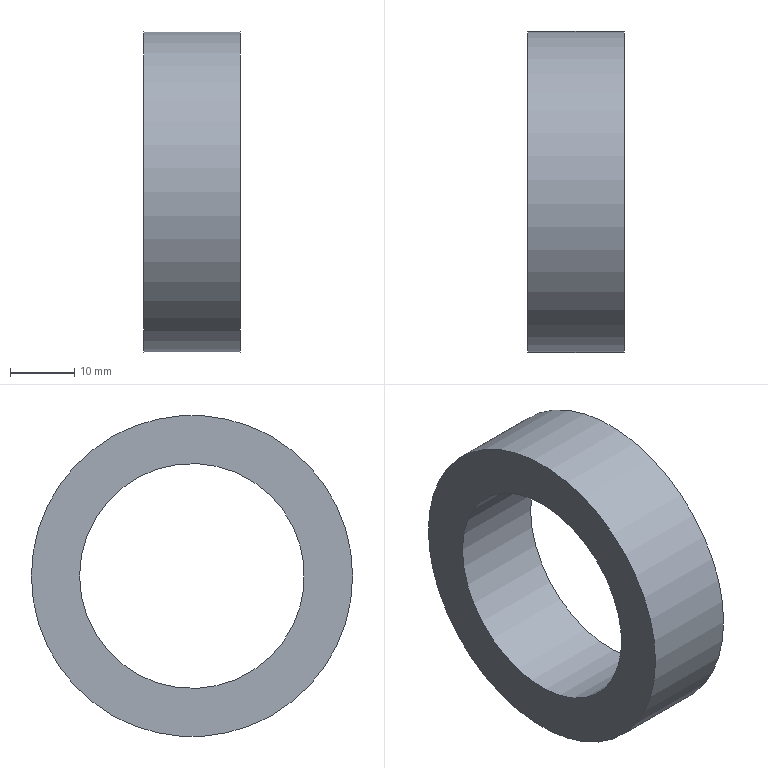Component | NX | CHENTAO | 1 solid | 4 faces | box 15 x 50 x 50 mm | volume 15021 mm3 | cylinder 2 | plane 2 | commonest cylinder face diameters 50 x1 35 x1
STEP:
#1=CARTESIAN_POINT('',(0.,0.,0.));
#2=DIRECTION('',(0.,0.,1.));
#3=DIRECTION('',(1.,0.,0.));
#4=AXIS2_PLACEMENT_3D('',#1,#2,#3);
#5=CARTESIAN_POINT('',(70.25,225.,-88.));
#6=VERTEX_POINT('',#5);
#7=CARTESIAN_POINT('',(70.25,200.,-88.));
#8=DIRECTION('',(1.,0.,0.));
#9=DIRECTION('',(0.,1.,0.));
#10=AXIS2_PLACEMENT_3D('',#7,#8,#9);
#11=CIRCLE('',#10,25.);
#12=CARTESIAN_POINT('',(70.25,200.,-88.));
#13=DIRECTION('',(-1.,0.,0.));
#14=DIRECTION('',(0.,0.,1.));
#15=AXIS2_PLACEMENT_3D('',#12,#13,#14);
#16=CYLINDRICAL_SURFACE('',#15,25.);
#17=CARTESIAN_POINT('',(7.854,0.));
#18=DIRECTION('',(-1.,0.));
#19=VECTOR('',#18,1.);
#20=LINE('',#17,#19);
#21=(GEOMETRIC_REPRESENTATION_CONTEXT(2)PARAMETRIC_REPRESENTATION_CONTEXT()REPRESENTATION_CONTEXT('',''));
#22=DEFINITIONAL_REPRESENTATION('',(#20),#21);
#23=PCURVE('',#16,#22);
#24=CARTESIAN_POINT('',(70.25,200.,-88.));
#25=DIRECTION('',(1.,0.,0.));
#26=DIRECTION('',(0.,0.,-1.));
#27=AXIS2_PLACEMENT_3D('',#24,#25,#26);
#28=PLANE('',#27);
#29=CARTESIAN_POINT('',(0.,0.));
#30=DIRECTION('',(0.,1.));
#31=AXIS2_PLACEMENT_2D('',#29,#30);
#32=CIRCLE('',#31,25.);
#33=(GEOMETRIC_REPRESENTATION_CONTEXT(2)PARAMETRIC_REPRESENTATION_CONTEXT()REPRESENTATION_CONTEXT('',''));
#34=DEFINITIONAL_REPRESENTATION('',(#32),#33);
#35=PCURVE('',#28,#34);
#36=SURFACE_CURVE('',#11,(#23,#35),.PCURVE_S1.);
#37=EDGE_CURVE('',#6,#6,#36,.T.);
#38=ORIENTED_EDGE('',*,*,#37,.F.);
#39=CARTESIAN_POINT('',(55.25,225.,-88.));
#40=VERTEX_POINT('',#39);
#41=CARTESIAN_POINT('',(70.25,225.,-88.));
#42=CARTESIAN_POINT('',(55.25,225.,-88.));
#43=B_SPLINE_CURVE_WITH_KNOTS('',1,(#41,#42),.UNSPECIFIED.,.F.,.F.,(2,2),(0.,15.),.PIECEWISE_BEZIER_KNOTS.);
#44=CARTESIAN_POINT('',(7.854,0.));
#45=DIRECTION('',(0.,1.));
#46=VECTOR('',#45,1.);
#47=LINE('',#44,#46);
#48=(GEOMETRIC_REPRESENTATION_CONTEXT(2)PARAMETRIC_REPRESENTATION_CONTEXT()REPRESENTATION_CONTEXT('',''));
#49=DEFINITIONAL_REPRESENTATION('',(#47),#48);
#50=PCURVE('',#16,#49);
#51=CARTESIAN_POINT('',(1.571,0.));
#52=DIRECTION('',(0.,1.));
#53=VECTOR('',#52,1.);
#54=LINE('',#51,#53);
#55=(GEOMETRIC_REPRESENTATION_CONTEXT(2)PARAMETRIC_REPRESENTATION_CONTEXT()REPRESENTATION_CONTEXT('',''));
#56=DEFINITIONAL_REPRESENTATION('',(#54),#55);
#57=PCURVE('',#16,#56);
#58=SEAM_CURVE('',#43,(#50,#57),.PCURVE_S1.);
#59=EDGE_CURVE('',#6,#40,#58,.T.);
#60=ORIENTED_EDGE('',*,*,#59,.T.);
#61=CARTESIAN_POINT('',(55.25,200.,-88.));
#62=DIRECTION('',(1.,0.,0.));
#63=DIRECTION('',(0.,1.,0.));
#64=AXIS2_PLACEMENT_3D('',#61,#62,#63);
#65=CIRCLE('',#64,25.);
#66=CARTESIAN_POINT('',(7.854,15.));
#67=DIRECTION('',(-1.,0.));
#68=VECTOR('',#67,1.);
#69=LINE('',#66,#68);
#70=(GEOMETRIC_REPRESENTATION_CONTEXT(2)PARAMETRIC_REPRESENTATION_CONTEXT()REPRESENTATION_CONTEXT('',''));
#71=DEFINITIONAL_REPRESENTATION('',(#69),#70);
#72=PCURVE('',#16,#71);
#73=CARTESIAN_POINT('',(55.25,200.,-88.));
#74=DIRECTION('',(1.,0.,0.));
#75=DIRECTION('',(0.,0.,-1.));
#76=AXIS2_PLACEMENT_3D('',#73,#74,#75);
#77=PLANE('',#76);
#78=CARTESIAN_POINT('',(0.,0.));
#79=DIRECTION('',(0.,1.));
#80=AXIS2_PLACEMENT_2D('',#78,#79);
#81=CIRCLE('',#80,25.);
#82=(GEOMETRIC_REPRESENTATION_CONTEXT(2)PARAMETRIC_REPRESENTATION_CONTEXT()REPRESENTATION_CONTEXT('',''));
#83=DEFINITIONAL_REPRESENTATION('',(#81),#82);
#84=PCURVE('',#77,#83);
#85=SURFACE_CURVE('',#65,(#72,#84),.PCURVE_S1.);
#86=EDGE_CURVE('',#40,#40,#85,.T.);
#87=ORIENTED_EDGE('',*,*,#86,.T.);
#88=ORIENTED_EDGE('',*,*,#59,.F.);
#89=EDGE_LOOP('',(#38,#60,#87,#88));
#90=FACE_BOUND('',#89,.T.);
#91=ADVANCED_FACE('',(#90),#16,.T.);
#92=CARTESIAN_POINT('',(70.25,217.5,-88.));
#93=VERTEX_POINT('',#92);
#94=CARTESIAN_POINT('',(70.25,200.,-88.));
#95=DIRECTION('',(1.,0.,0.));
#96=DIRECTION('',(0.,1.,0.));
#97=AXIS2_PLACEMENT_3D('',#94,#95,#96);
#98=CIRCLE('',#97,17.5);
#99=CARTESIAN_POINT('',(70.25,200.,-88.));
#100=DIRECTION('',(-1.,0.,0.));
#101=DIRECTION('',(0.,0.,1.));
#102=AXIS2_PLACEMENT_3D('',#99,#100,#101);
#103=CYLINDRICAL_SURFACE('',#102,17.5);
#104=CARTESIAN_POINT('',(7.854,0.));
#105=DIRECTION('',(-1.,0.));
#106=VECTOR('',#105,1.);
#107=LINE('',#104,#106);
#108=(GEOMETRIC_REPRESENTATION_CONTEXT(2)PARAMETRIC_REPRESENTATION_CONTEXT()REPRESENTATION_CONTEXT('',''));
#109=DEFINITIONAL_REPRESENTATION('',(#107),#108);
#110=PCURVE('',#103,#109);
#111=CARTESIAN_POINT('',(0.,0.));
#112=DIRECTION('',(0.,1.));
#113=AXIS2_PLACEMENT_2D('',#111,#112);
#114=CIRCLE('',#113,17.5);
#115=(GEOMETRIC_REPRESENTATION_CONTEXT(2)PARAMETRIC_REPRESENTATION_CONTEXT()REPRESENTATION_CONTEXT('',''));
#116=DEFINITIONAL_REPRESENTATION('',(#114),#115);
#117=PCURVE('',#28,#116);
#118=SURFACE_CURVE('',#98,(#110,#117),.PCURVE_S1.);
#119=EDGE_CURVE('',#93,#93,#118,.T.);
#120=ORIENTED_EDGE('',*,*,#119,.F.);
#121=CARTESIAN_POINT('',(55.25,217.5,-88.));
#122=VERTEX_POINT('',#121);
#123=CARTESIAN_POINT('',(70.25,217.5,-88.));
#124=CARTESIAN_POINT('',(55.25,217.5,-88.));
#125=B_SPLINE_CURVE_WITH_KNOTS('',1,(#123,#124),.UNSPECIFIED.,.F.,.F.,(2,2),(0.,15.),.PIECEWISE_BEZIER_KNOTS.);
#126=CARTESIAN_POINT('',(7.854,0.));
#127=DIRECTION('',(0.,1.));
#128=VECTOR('',#127,1.);
#129=LINE('',#126,#128);
#130=(GEOMETRIC_REPRESENTATION_CONTEXT(2)PARAMETRIC_REPRESENTATION_CONTEXT()REPRESENTATION_CONTEXT('',''));
#131=DEFINITIONAL_REPRESENTATION('',(#129),#130);
#132=PCURVE('',#103,#131);
#133=CARTESIAN_POINT('',(1.571,0.));
#134=DIRECTION('',(0.,1.));
#135=VECTOR('',#134,1.);
#136=LINE('',#133,#135);
#137=(GEOMETRIC_REPRESENTATION_CONTEXT(2)PARAMETRIC_REPRESENTATION_CONTEXT()REPRESENTATION_CONTEXT('',''));
#138=DEFINITIONAL_REPRESENTATION('',(#136),#137);
#139=PCURVE('',#103,#138);
#140=SEAM_CURVE('',#125,(#132,#139),.PCURVE_S1.);
#141=EDGE_CURVE('',#93,#122,#140,.T.);
#142=ORIENTED_EDGE('',*,*,#141,.T.);
#143=CARTESIAN_POINT('',(55.25,200.,-88.));
#144=DIRECTION('',(1.,0.,0.));
#145=DIRECTION('',(0.,1.,0.));
#146=AXIS2_PLACEMENT_3D('',#143,#144,#145);
#147=CIRCLE('',#146,17.5);
#148=CARTESIAN_POINT('',(7.854,15.));
#149=DIRECTION('',(-1.,0.));
#150=VECTOR('',#149,1.);
#151=LINE('',#148,#150);
#152=(GEOMETRIC_REPRESENTATION_CONTEXT(2)PARAMETRIC_REPRESENTATION_CONTEXT()REPRESENTATION_CONTEXT('',''));
#153=DEFINITIONAL_REPRESENTATION('',(#151),#152);
#154=PCURVE('',#103,#153);
#155=CARTESIAN_POINT('',(0.,0.));
#156=DIRECTION('',(0.,1.));
#157=AXIS2_PLACEMENT_2D('',#155,#156);
#158=CIRCLE('',#157,17.5);
#159=(GEOMETRIC_REPRESENTATION_CONTEXT(2)PARAMETRIC_REPRESENTATION_CONTEXT()REPRESENTATION_CONTEXT('',''));
#160=DEFINITIONAL_REPRESENTATION('',(#158),#159);
#161=PCURVE('',#77,#160);
#162=SURFACE_CURVE('',#147,(#154,#161),.PCURVE_S1.);
#163=EDGE_CURVE('',#122,#122,#162,.T.);
#164=ORIENTED_EDGE('',*,*,#163,.T.);
#165=ORIENTED_EDGE('',*,*,#141,.F.);
#166=EDGE_LOOP('',(#120,#142,#164,#165));
#167=FACE_BOUND('',#166,.F.);
#168=ADVANCED_FACE('',(#167),#103,.F.);
#169=ORIENTED_EDGE('',*,*,#37,.T.);
#170=EDGE_LOOP('',(#169));
#171=FACE_BOUND('',#170,.T.);
#172=ORIENTED_EDGE('',*,*,#119,.F.);
#173=EDGE_LOOP('',(#172));
#174=FACE_BOUND('',#173,.T.);
#175=ADVANCED_FACE('',(#171,#174),#28,.T.);
#176=ORIENTED_EDGE('',*,*,#86,.F.);
#177=EDGE_LOOP('',(#176));
#178=FACE_BOUND('',#177,.T.);
#179=ORIENTED_EDGE('',*,*,#163,.T.);
#180=EDGE_LOOP('',(#179));
#181=FACE_BOUND('',#180,.T.);
#182=ADVANCED_FACE('',(#178,#181),#77,.F.);
#183=CLOSED_SHELL('',(#91,#168,#175,#182));
#184=MANIFOLD_SOLID_BREP('',#183);
#185=(LENGTH_UNIT()NAMED_UNIT(*)SI_UNIT(.MILLI.,.METRE.));
#186=UNCERTAINTY_MEASURE_WITH_UNIT(LENGTH_MEASURE(0.00001),#185,'','');
#187=(NAMED_UNIT(*)PLANE_ANGLE_UNIT()SI_UNIT($,.RADIAN.));
#188=(NAMED_UNIT(*)SI_UNIT($,.STERADIAN.)SOLID_ANGLE_UNIT());
#189=(GEOMETRIC_REPRESENTATION_CONTEXT(3)GLOBAL_UNCERTAINTY_ASSIGNED_CONTEXT((#186))GLOBAL_UNIT_ASSIGNED_CONTEXT((#185,#187,#188))REPRESENTATION_CONTEXT('',''));
#190=ADVANCED_BREP_SHAPE_REPRESENTATION('',(#4,#184),#189);